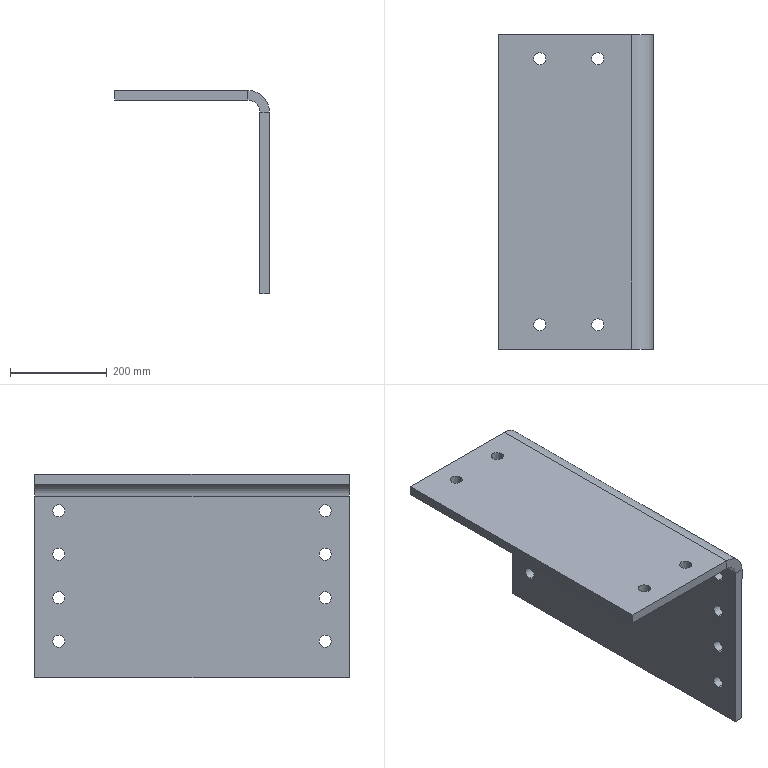Component | SolidWorks | Main-1_L-1 | 1 solid | 38 faces | volume 9046903 mm3 | cylinder 26 | plane 12 | commonest cylinder face diameters 25 x24 90 x1 50 x1 | material Plain Carbon Steel